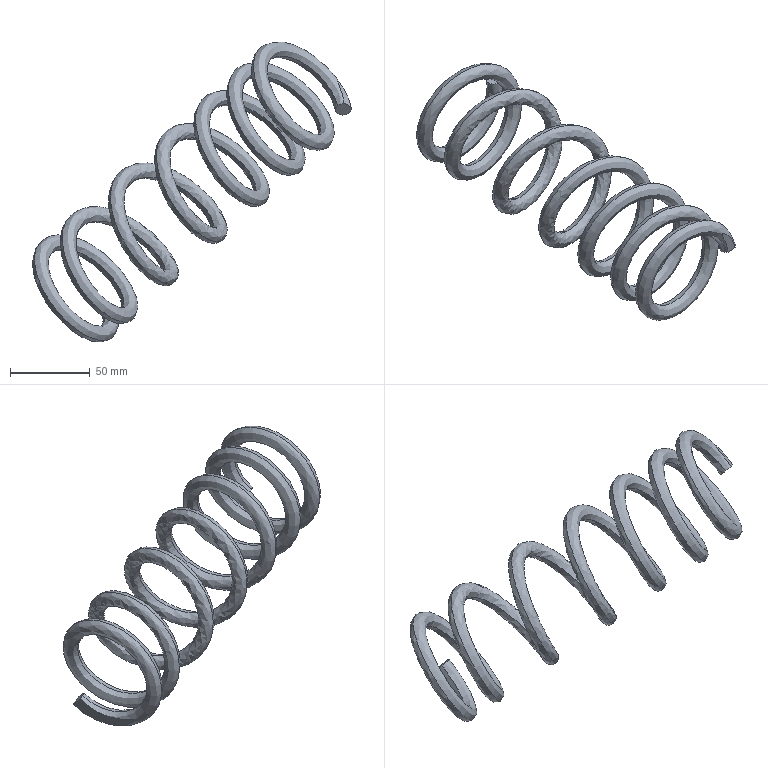Component | SolidWorks | BufferSpring2-1 | 1 solid | 6 faces | volume 112577 mm3 | plane 4 | spline 2 | material Chrome Stainless Steel